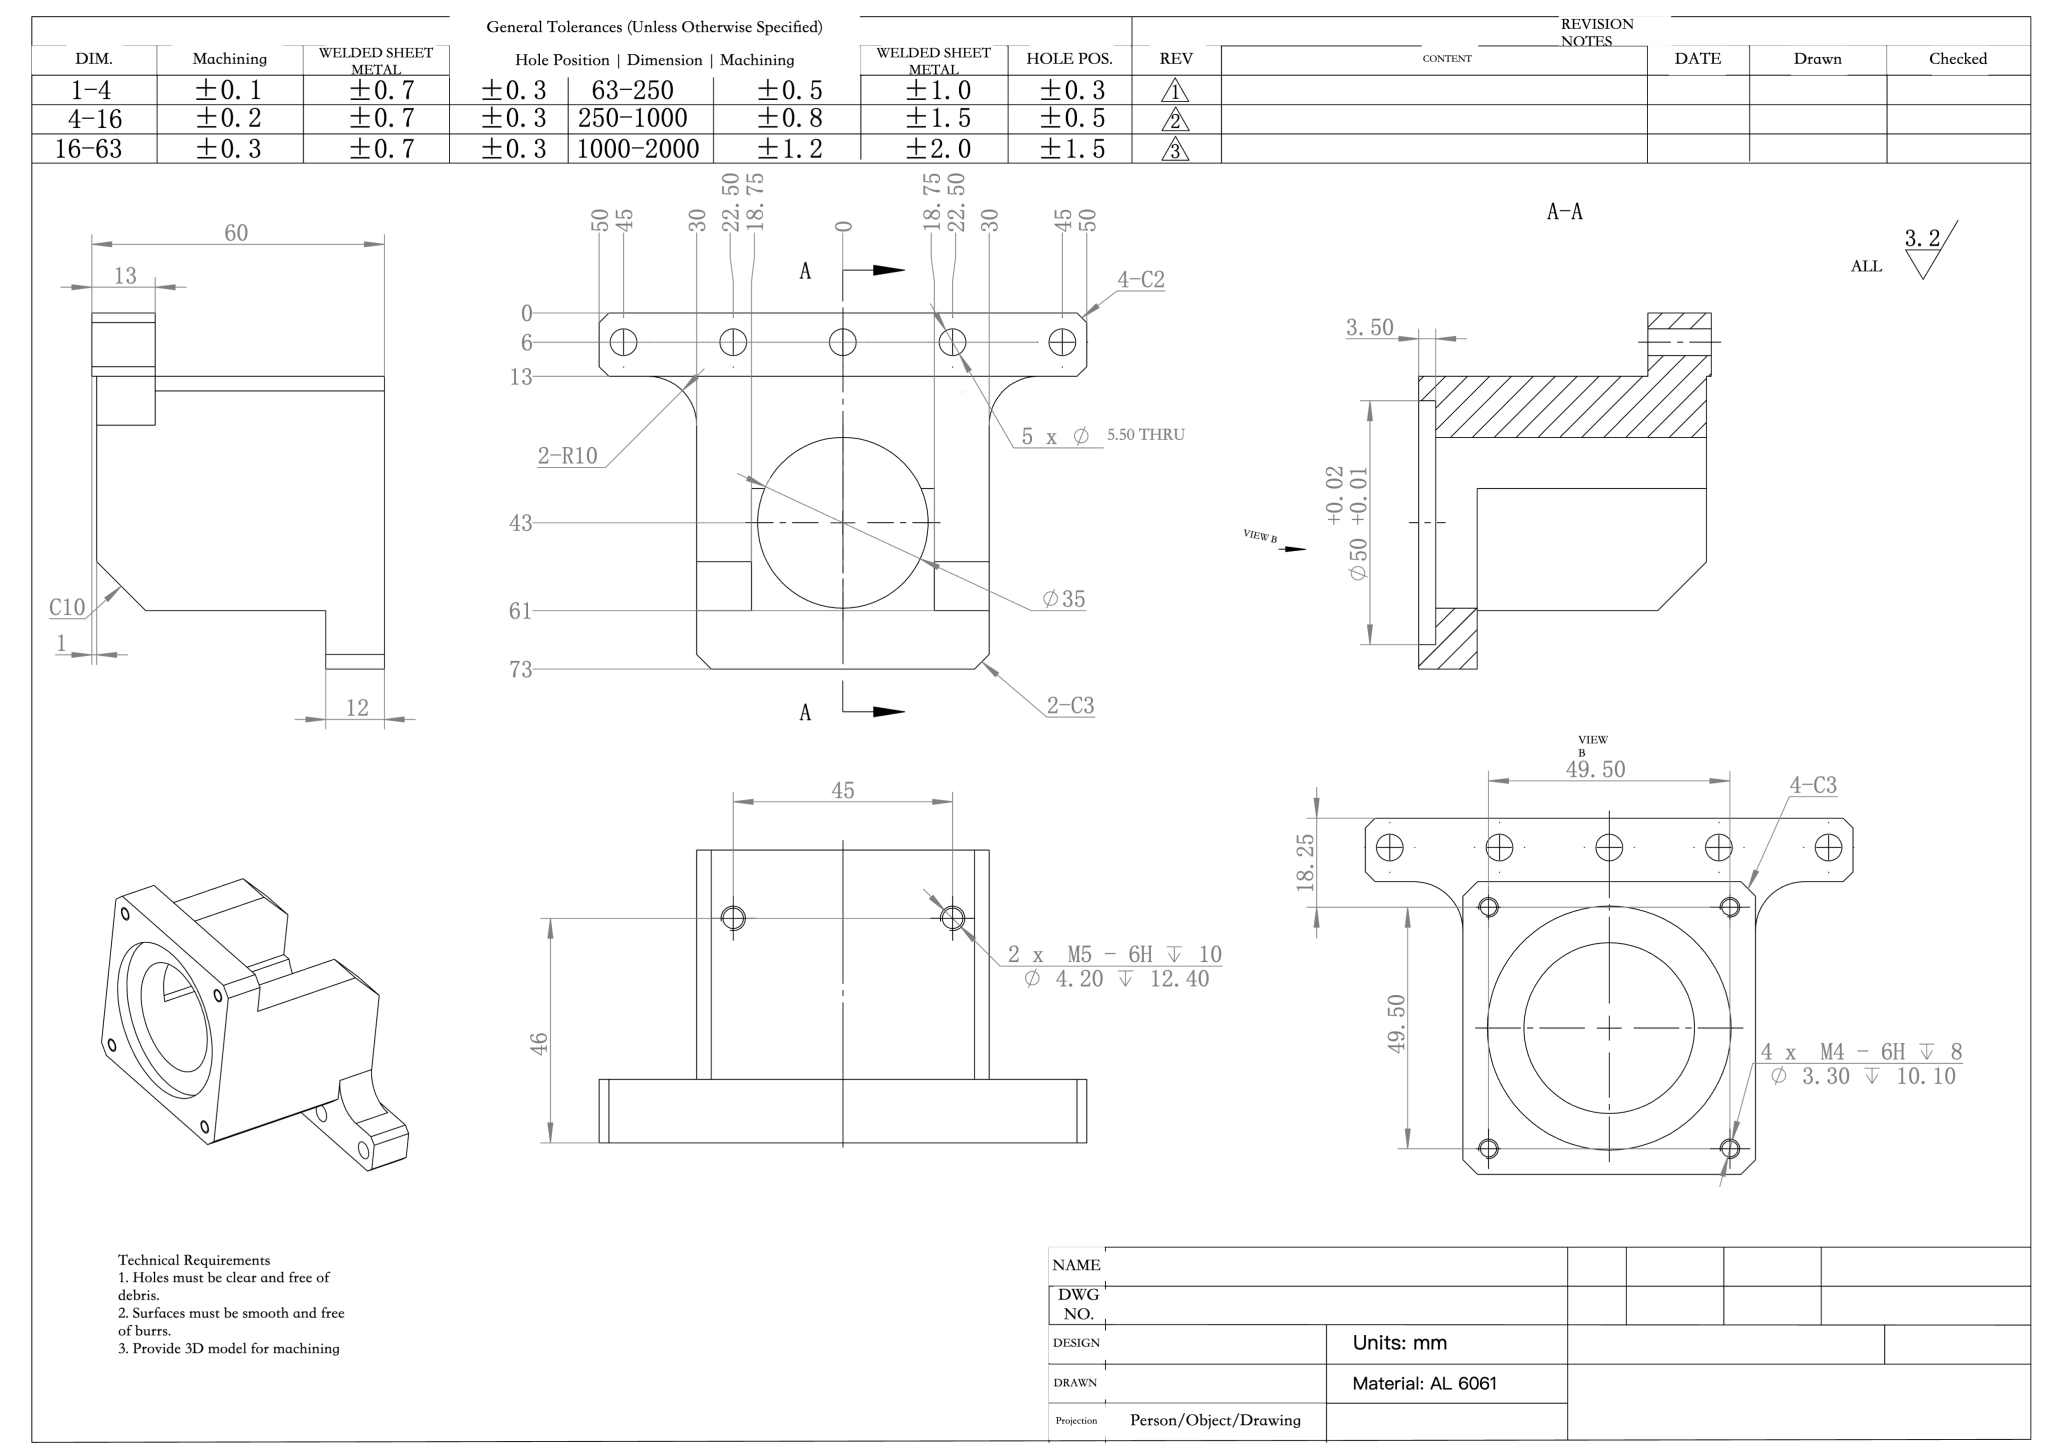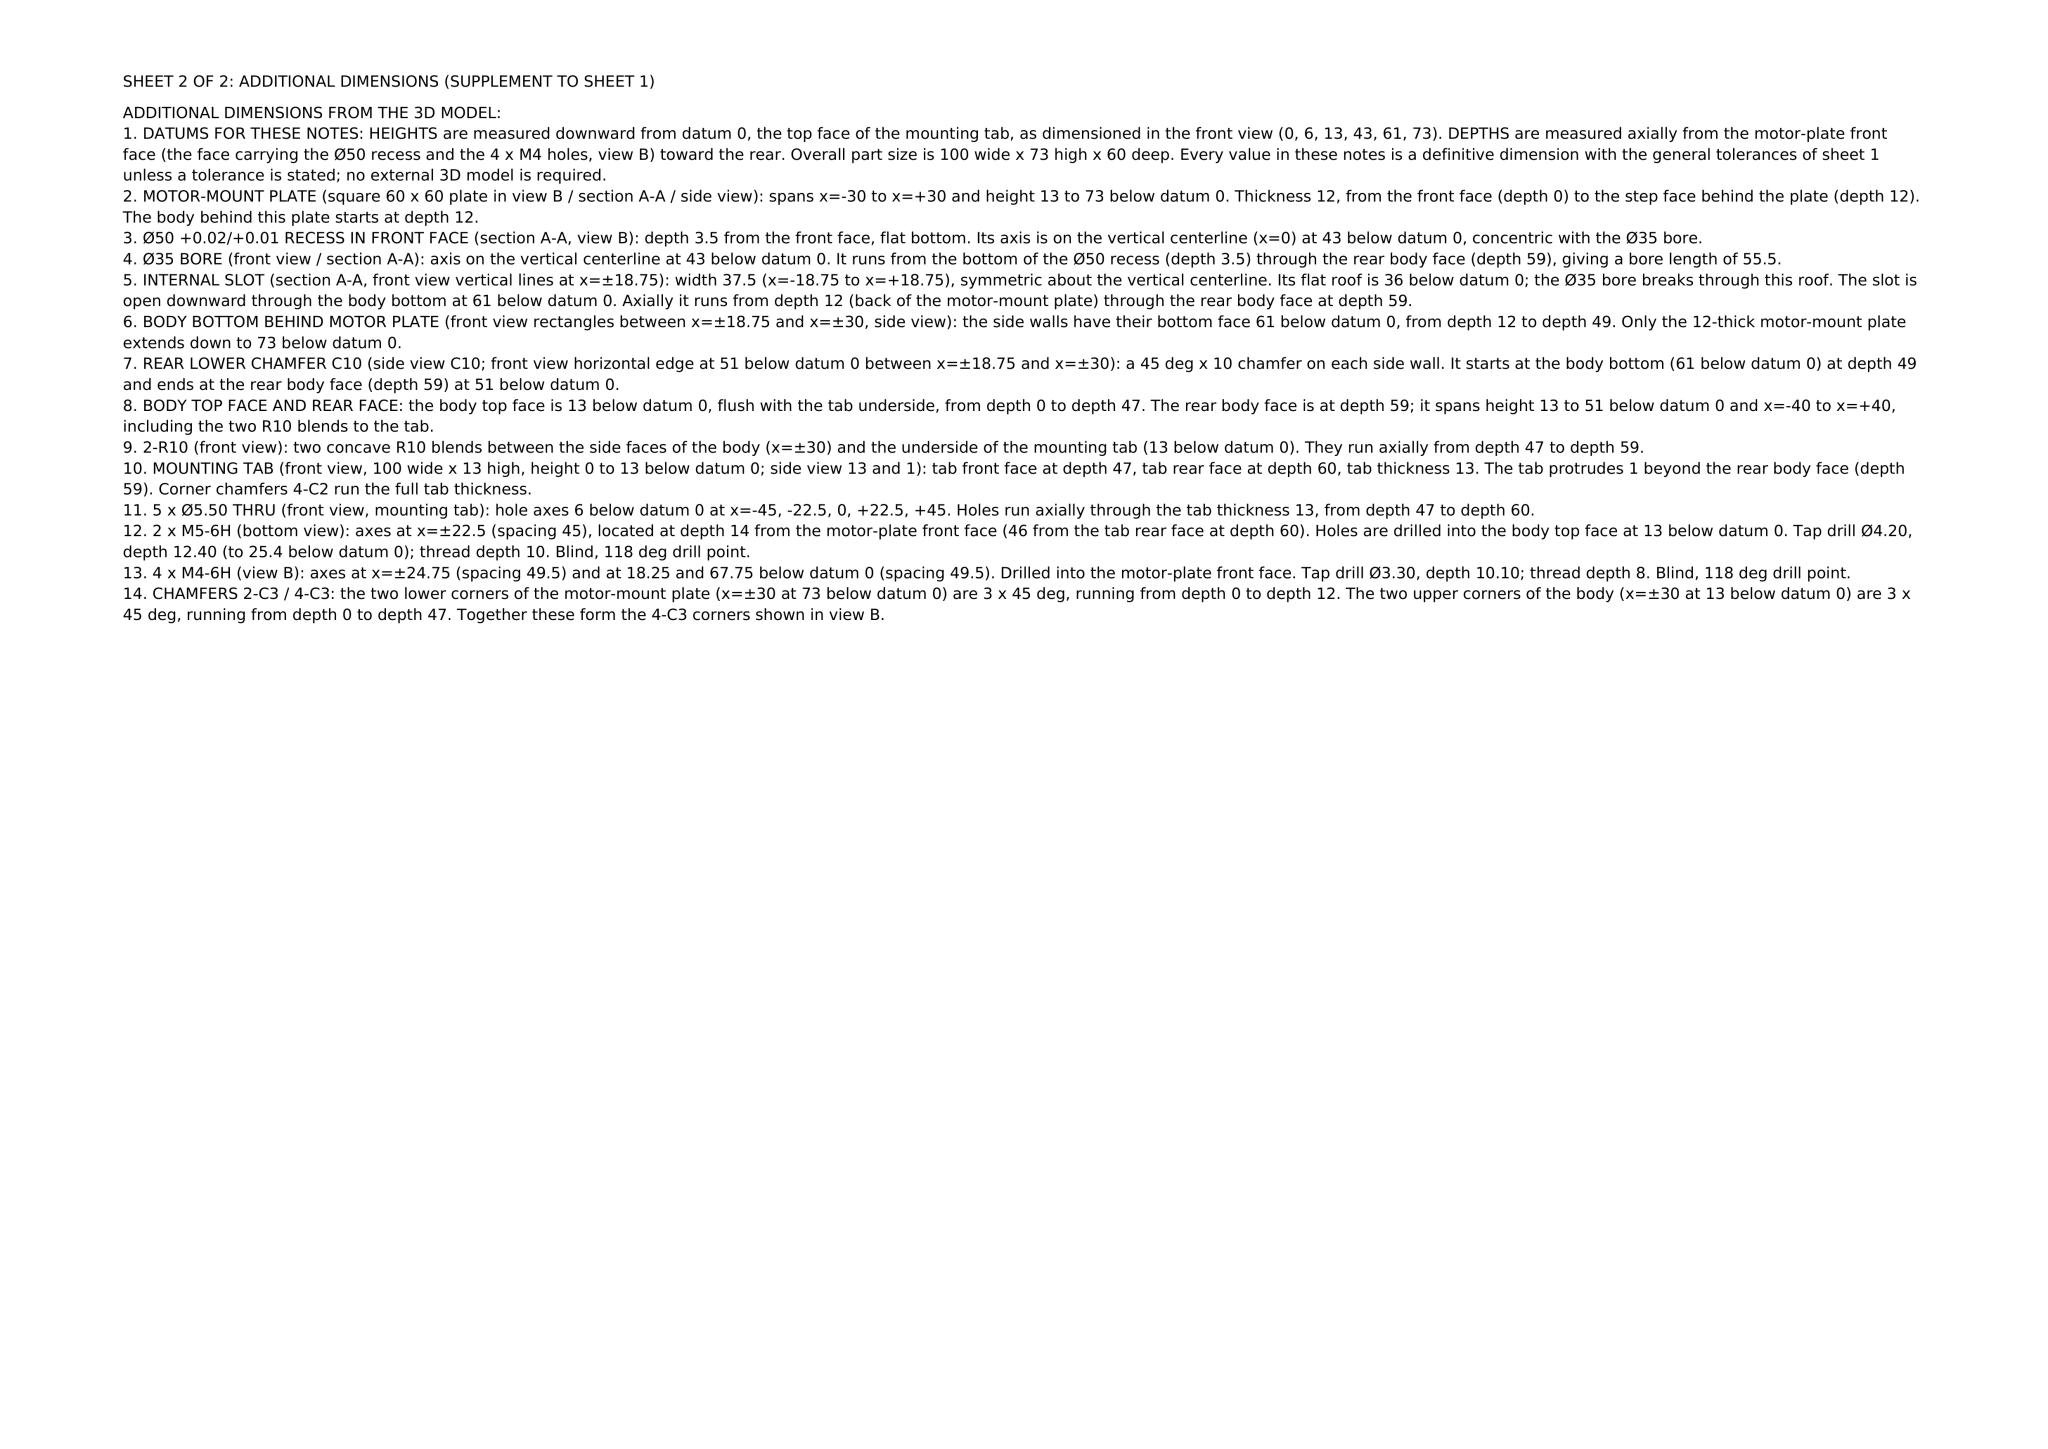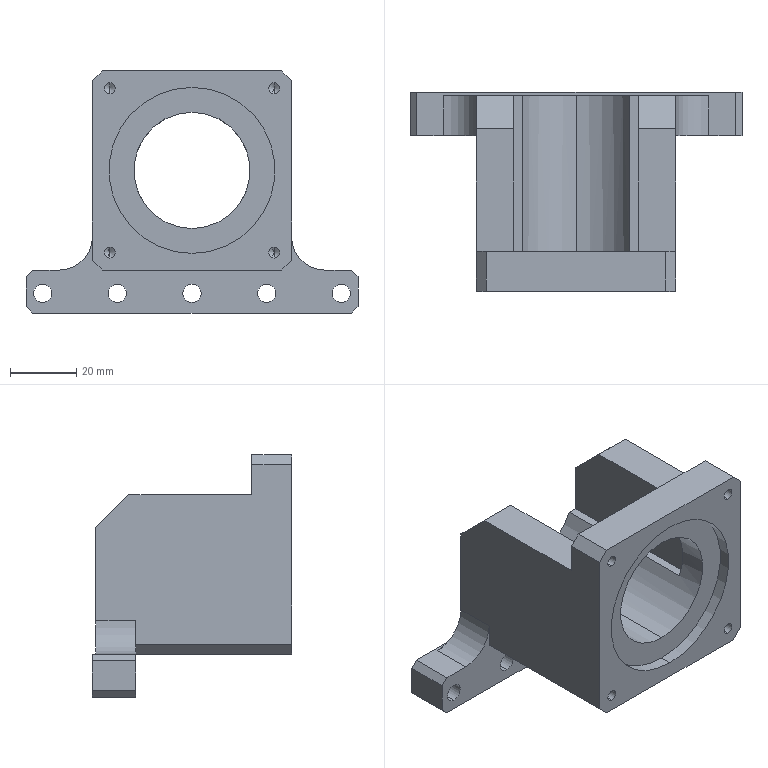Part | NX | mm | Stepped Bearing Mount Housing | 1 solid | 70 faces | box 100 x 60 x 73 mm | volume 121436 mm3 | plane 30 | cylinder 28 | cone 12 | commonest cylinder face diameters 5.5 x10 3.3 x8 4.2 x4 50 x2 35 x2 20 x2